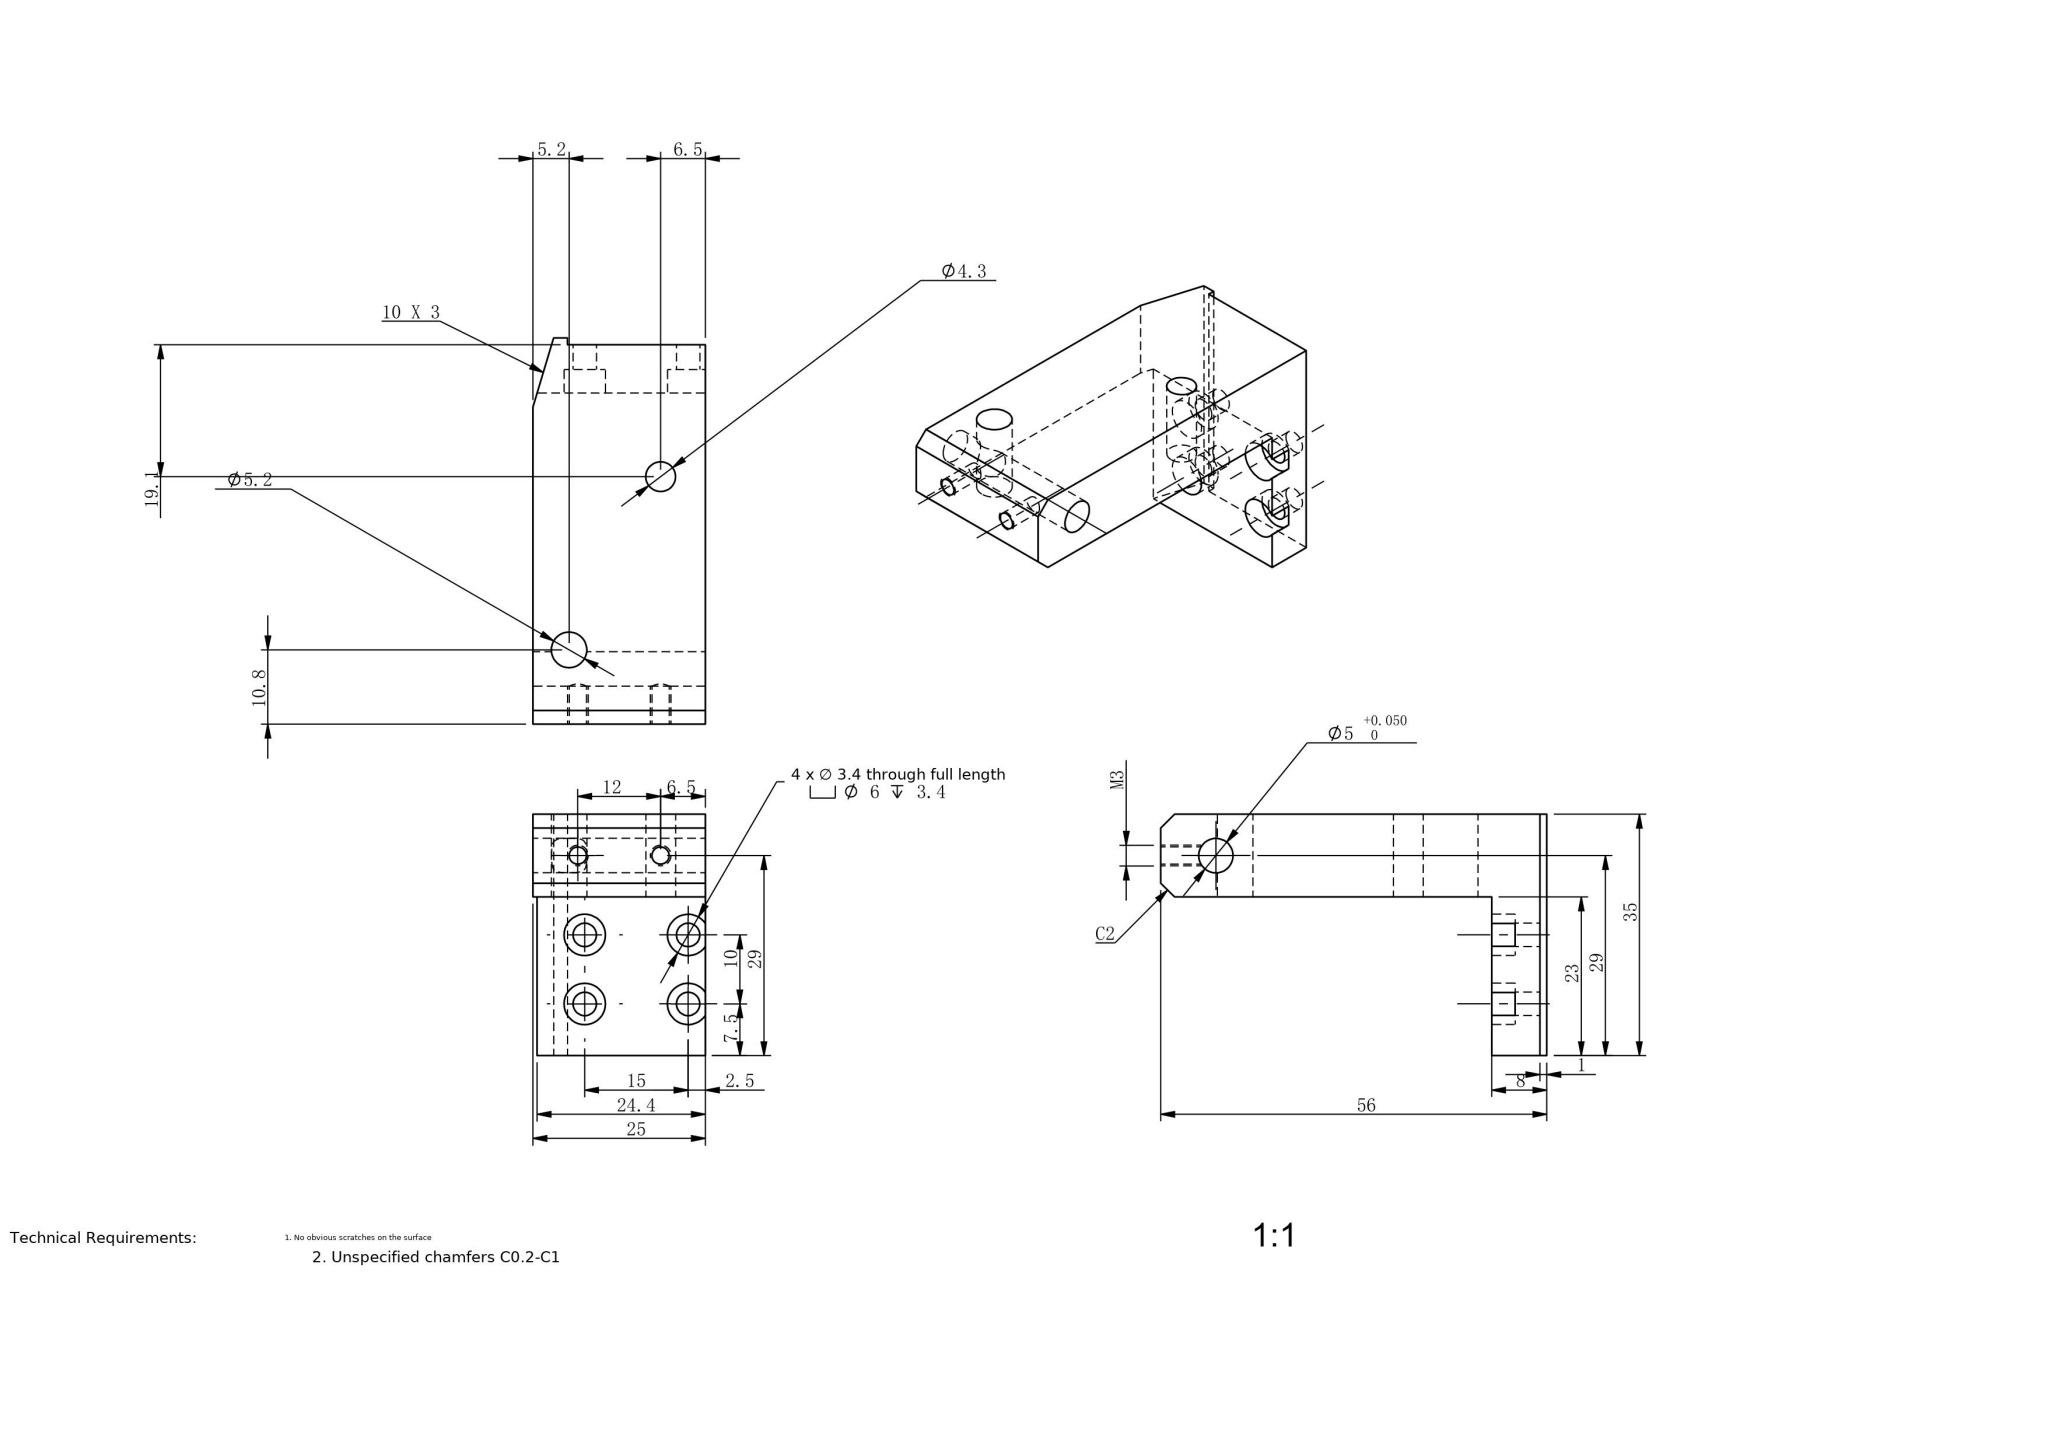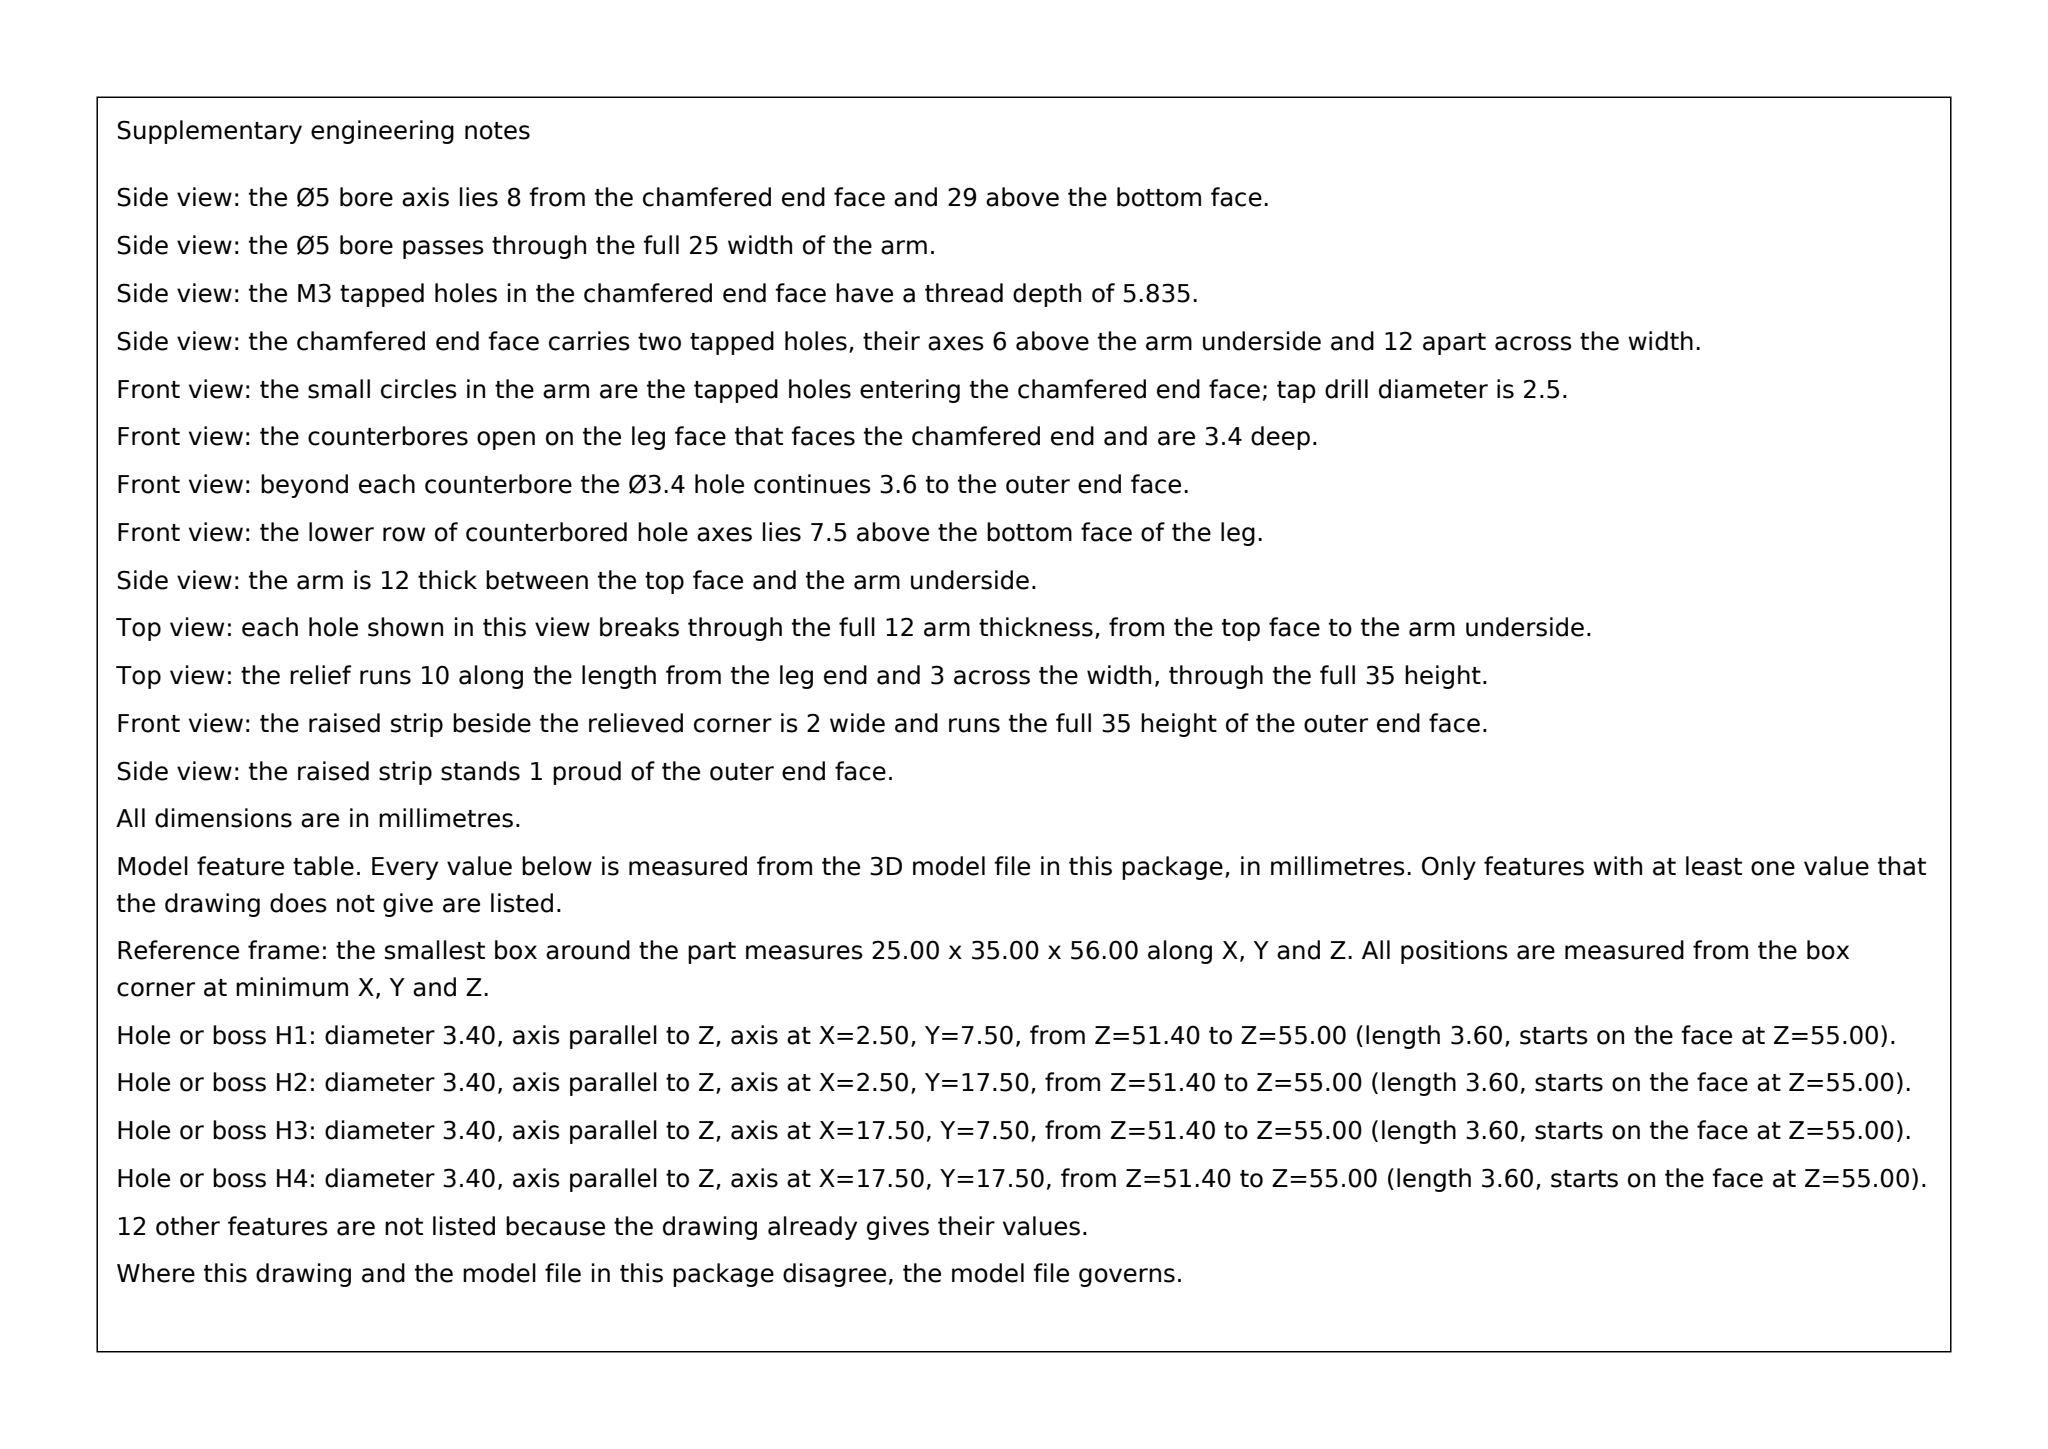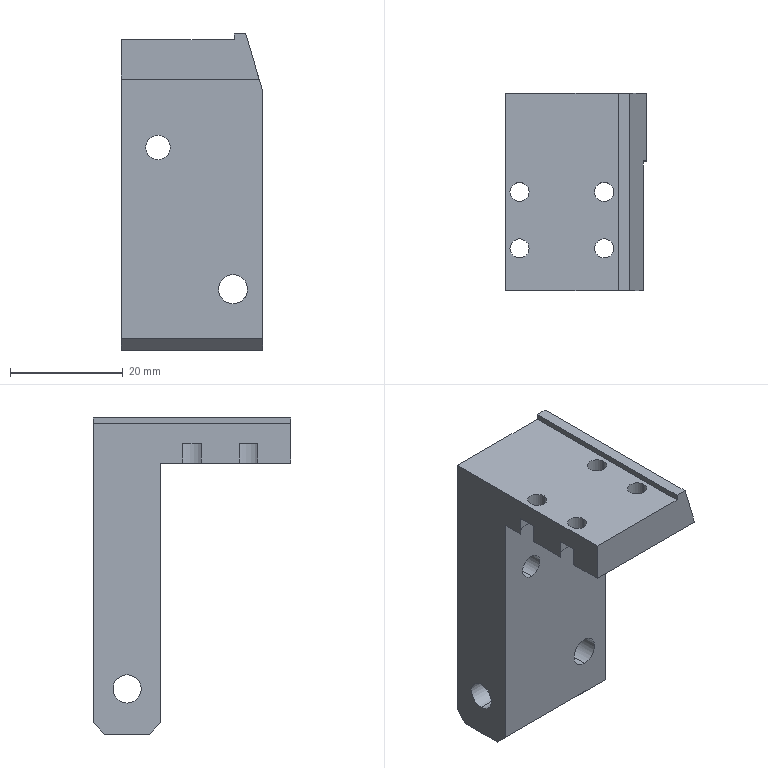Part | SolidWorks | mm | 1 solid | 41 faces | box 25 x 35 x 56 mm | volume 18641 mm3 | cylinder 24 | plane 17 | commonest cylinder face diameters 3.4 x8 6 x6 2.5 x4 4.32 x2 5.157 x2 5 x2
build123d program:
from build123d import *

# Parameters (mm, degrees)
SKETCH1_W                                            = 25
SKETCH1_H                                            = 56
BOSS_EXTRUDE1_DEPTH                                  = 35
SKETCH2_R                                            = 2.5
CUT_EXTRUDE1_DEPTH                                   = 30
SKETCH3_W                                            = 48
SKETCH3_H                                            = 23
CUT_EXTRUDE2_DEPTH                                   = 52.323
HOLE_SIZE_ACCORDING_TO_HEX_SOCKET_HEAD_C_D           = 3.4
HOLE_SIZE_ACCORDING_TO_HEX_SOCKET_HEAD_C_CBORE_D     = 6
HOLE_SIZE_ACCORDING_TO_HEX_SOCKET_HEAD_C_CBORE_DEPTH = 3.4
CHAMFER1_SIZE                                        = 3
CHAMFER1_SIZE2                                       = 10
SKETCH6_W                                            = 20
SKETCH6_H                                            = 55.203
CUT_EXTRUDE3_DEPTH                                   = 1
M3_TAPPED_HOLE1_D                                    = 2.5
M3_TAPPED_HOLE1_DEPTH                                = 8
M3_TAPPED_HOLE1_TIP                                  = 0.7511
CHAMFER2_SIZE                                        = 2
SKETCH9_R                                            = 2.16
SKETCH9_R_2                                          = 2.579
CUT_EXTRUDE4_DEPTH                                   = 41


with BuildPart() as part:
    # Sketch1 → Boss-Extrude1 (new body)
    with BuildSketch(Plane(origin=(0, 0, 0), x_dir=(1, 0, 0), z_dir=(0, 1, 0))):
        Rectangle(SKETCH1_W, SKETCH1_H)
    extrude(amount=BOSS_EXTRUDE1_DEPTH)

    # Sketch2 → Cut-Extrude1 (cut)
    with BuildSketch(Plane(origin=(12.5, 0, 0), x_dir=(0, 0, -1), z_dir=(1, 0, 0))):
        with Locations((20, 29)):
            Circle(SKETCH2_R)
    extrude(amount=-CUT_EXTRUDE1_DEPTH, mode=Mode.SUBTRACT)

    # Sketch3 → Cut-Extrude2 (cut, through all)
    with BuildSketch(Plane.ZY.offset(12.5)):
        with Locations((-4, 11.5)):
            Rectangle(SKETCH3_W, SKETCH3_H)
    extrude(amount=-CUT_EXTRUDE2_DEPTH, mode=Mode.SUBTRACT)

    # Hole Size according to Hex Socket Head C (through all)
    with Locations(Plane(origin=(0, 0, 20), x_dir=(-1, 0, 0), z_dir=(0, 0, -1))):
        with Locations((10, 17.5), (-5, 17.5), (-5, 7.5), (10, 7.5)):
            CounterBoreHole(HOLE_SIZE_ACCORDING_TO_HEX_SOCKET_HEAD_C_D / 2, HOLE_SIZE_ACCORDING_TO_HEX_SOCKET_HEAD_C_CBORE_D / 2, HOLE_SIZE_ACCORDING_TO_HEX_SOCKET_HEAD_C_CBORE_DEPTH)

    # Chamfer1
    chamfer1_edges = [part.edges().sort_by_distance(p)[0] for p in [
        (12.5, 17.5, 28),
    ]]
    chamfer1_side = [part.faces().sort_by_distance(p)[0] for p in [
        (0.1083, 17.717, 28),
    ]]
    chamfer(chamfer1_edges, length=CHAMFER1_SIZE, length2=CHAMFER1_SIZE2, reference=chamfer1_side[0])

    # Sketch6 → Cut-Extrude3 (cut)
    with BuildSketch(Plane.XY.offset(28)):
        with Locations((-2.5, 7.399)):
            Rectangle(SKETCH6_W, SKETCH6_H)
    extrude(amount=-CUT_EXTRUDE3_DEPTH, mode=Mode.SUBTRACT)

    # M3 Tapped Hole1
    with Locations(Plane(origin=(0, 0, -28), x_dir=(-1, 0, 0), z_dir=(0, 0, -1))):
        with Locations((6, 29), (-6, 29)):
            Hole(M3_TAPPED_HOLE1_D / 2, depth=M3_TAPPED_HOLE1_DEPTH)
            with Locations((0, 0, -(M3_TAPPED_HOLE1_DEPTH + M3_TAPPED_HOLE1_TIP / 2))):  # 118° drill point
                Cone(0, M3_TAPPED_HOLE1_D / 2, M3_TAPPED_HOLE1_TIP, mode=Mode.SUBTRACT)

    # Chamfer2
    chamfer2_edges = [part.edges().sort_by_distance(p)[0] for p in [
        (0, 23, -28),
        (0, 35, -28),
    ]]
    chamfer(chamfer2_edges, length=CHAMFER2_SIZE)

    # Sketch9 → Cut-Extrude4 (cut)
    with BuildSketch(Plane.XZ.offset(-23)):
        with Locations(Location((-6.025, 7.892, 0), (0, 0, 270))):
            Circle(SKETCH9_R)
        with Locations(Location((7.265, -17.222, 0), (0, 0, 270))):
            Circle(SKETCH9_R_2)
    extrude(amount=-CUT_EXTRUDE4_DEPTH, mode=Mode.SUBTRACT)


solid = part.part